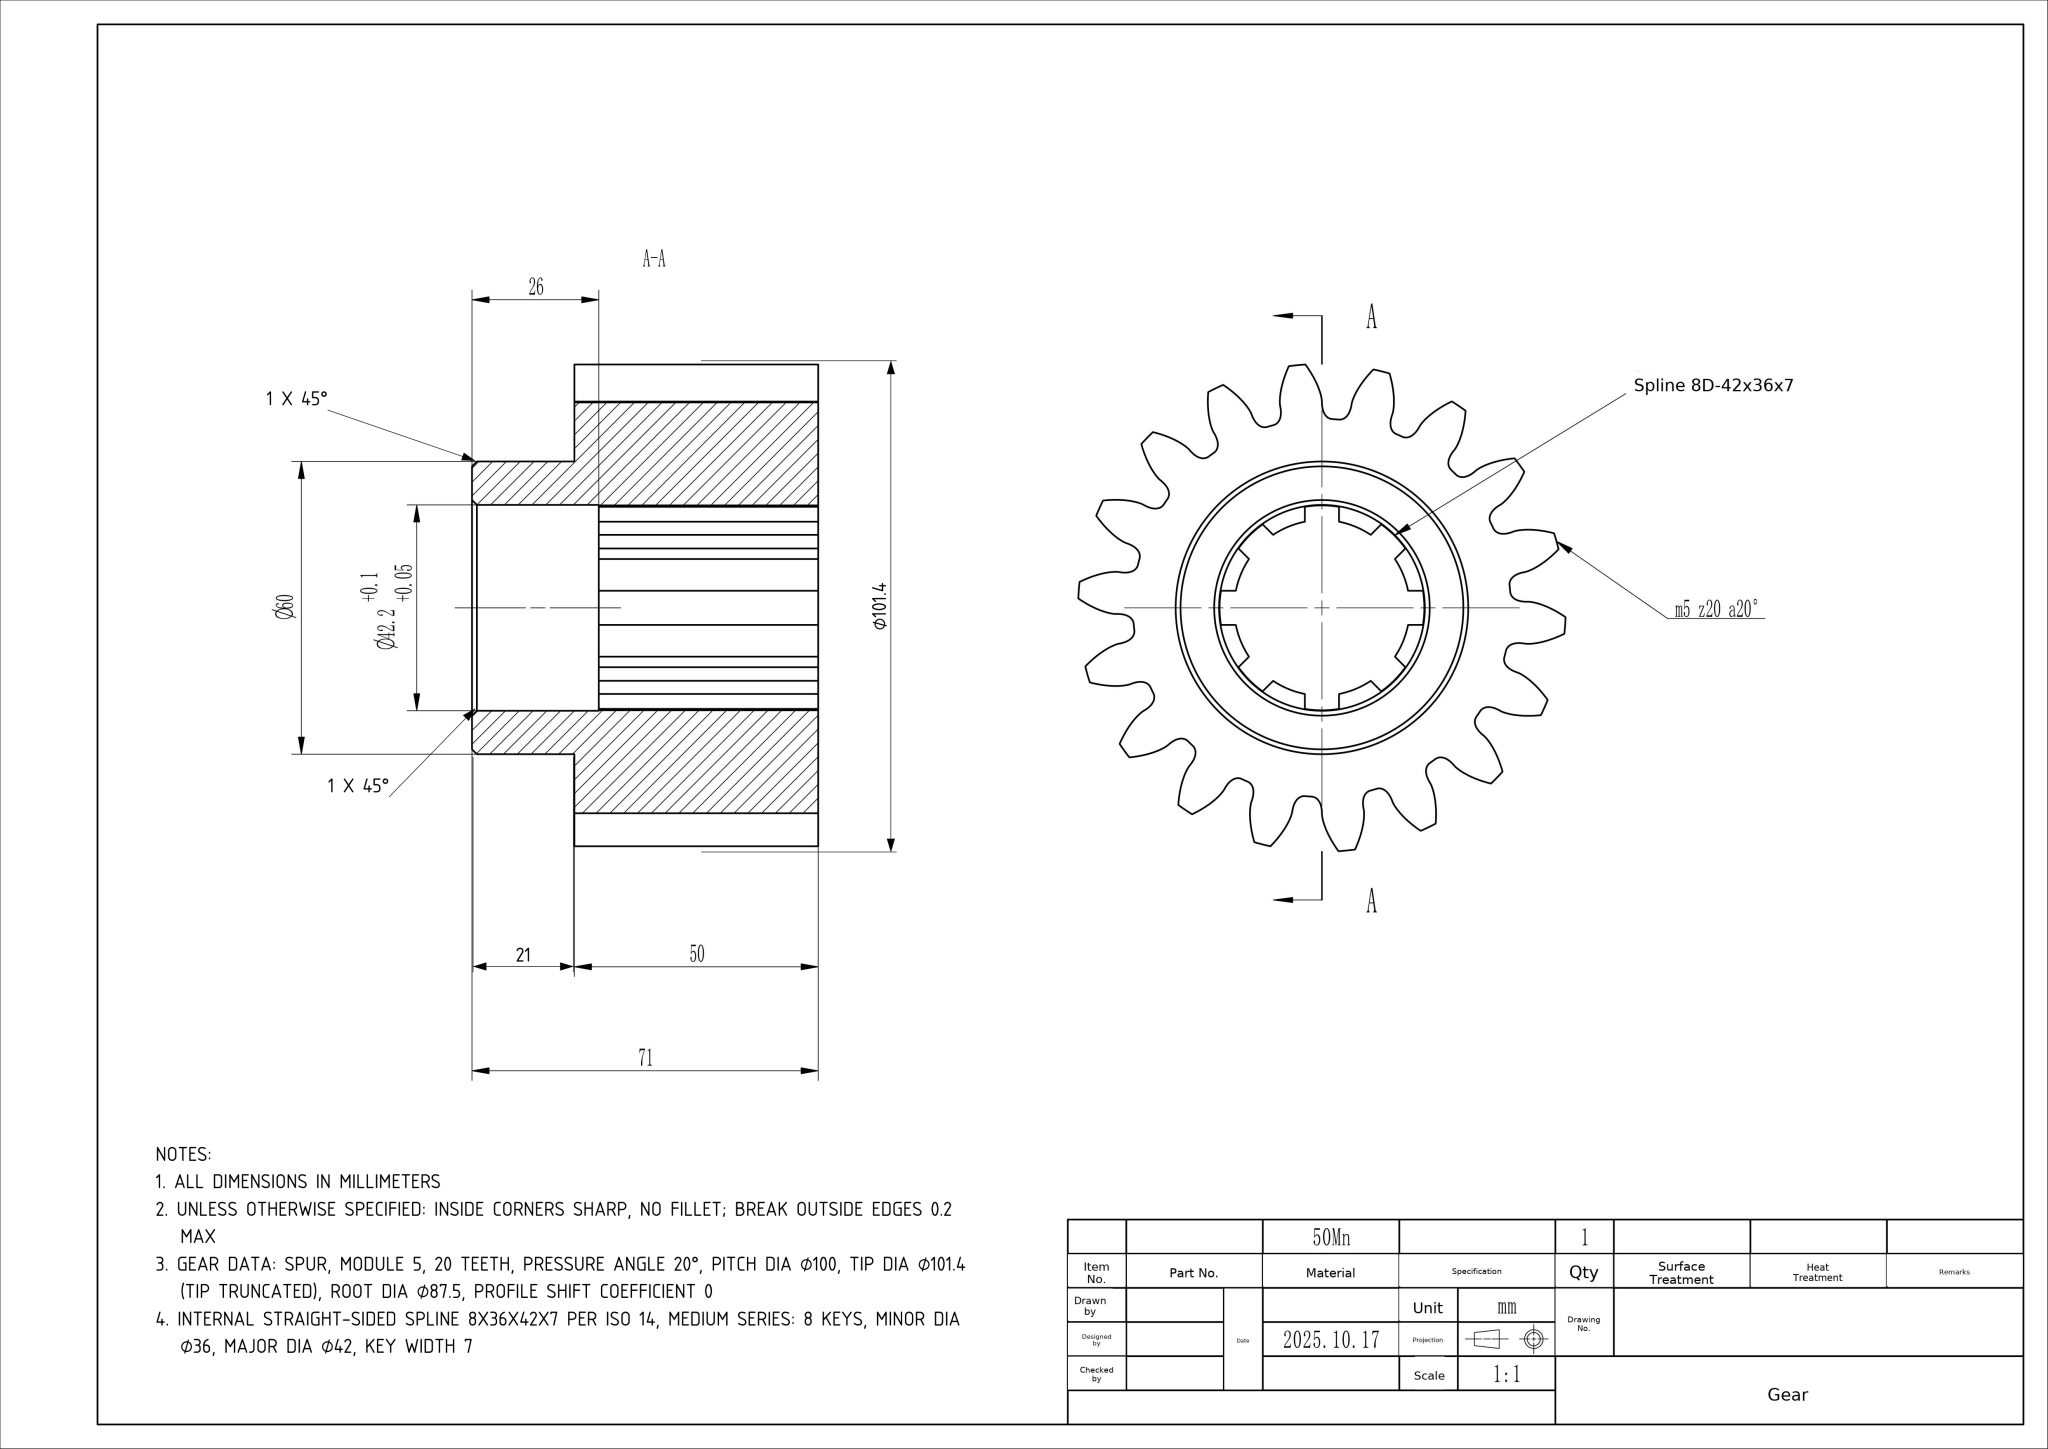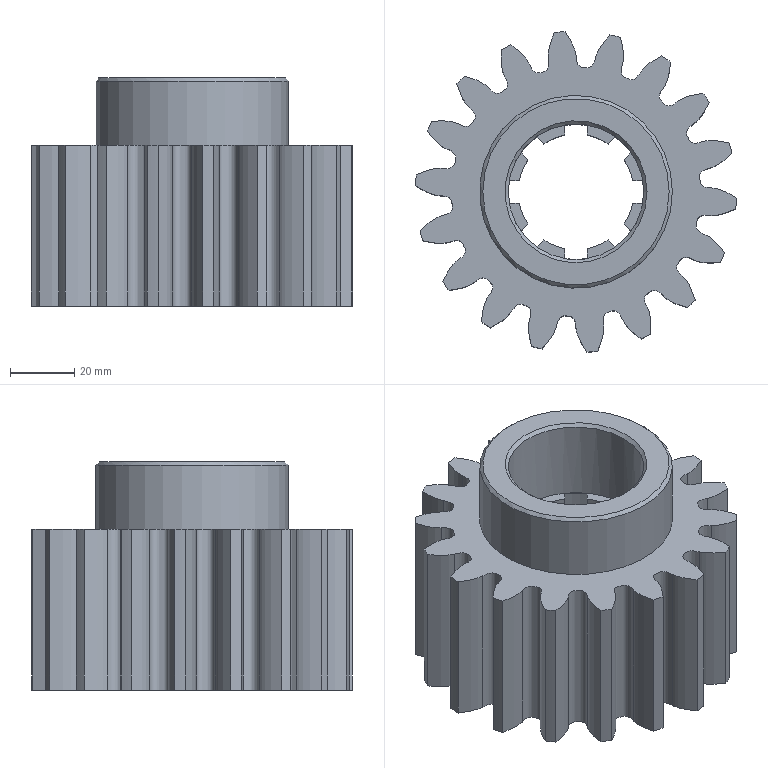Part | NX | mm | 1 solid | 112 faces | box 99.93 x 99.77 x 71 mm | volume 281767 mm3 | spline 54 | cylinder 36 | plane 20 | cone 2 | commonest cylinder face diameters 100 x18 42 x8 36 x8 60 x1 42.2 x1